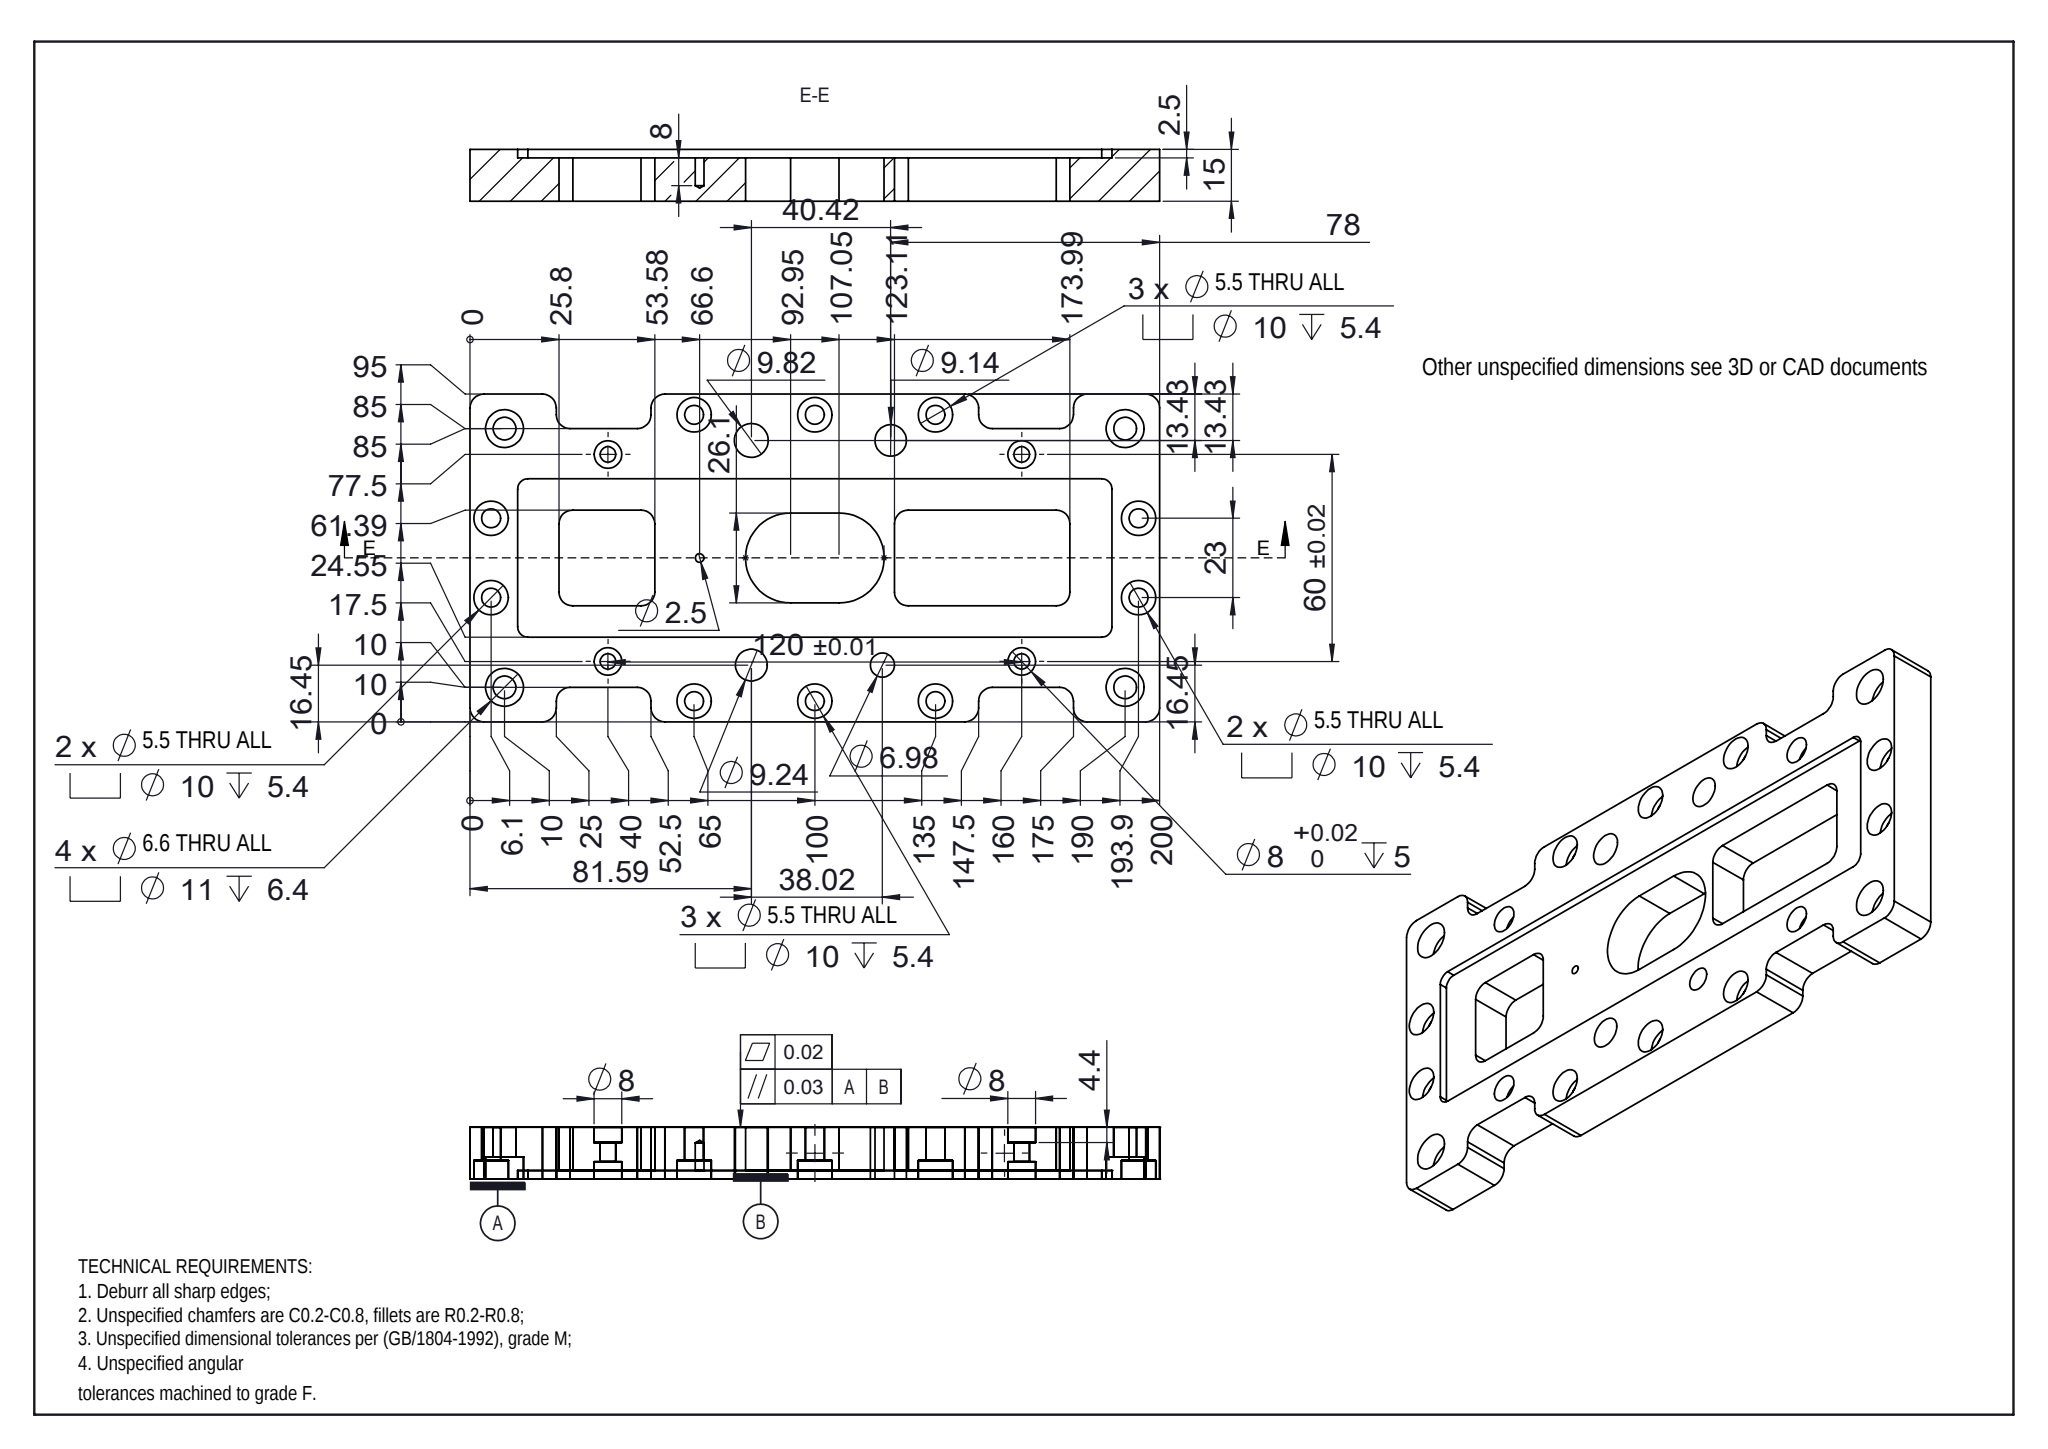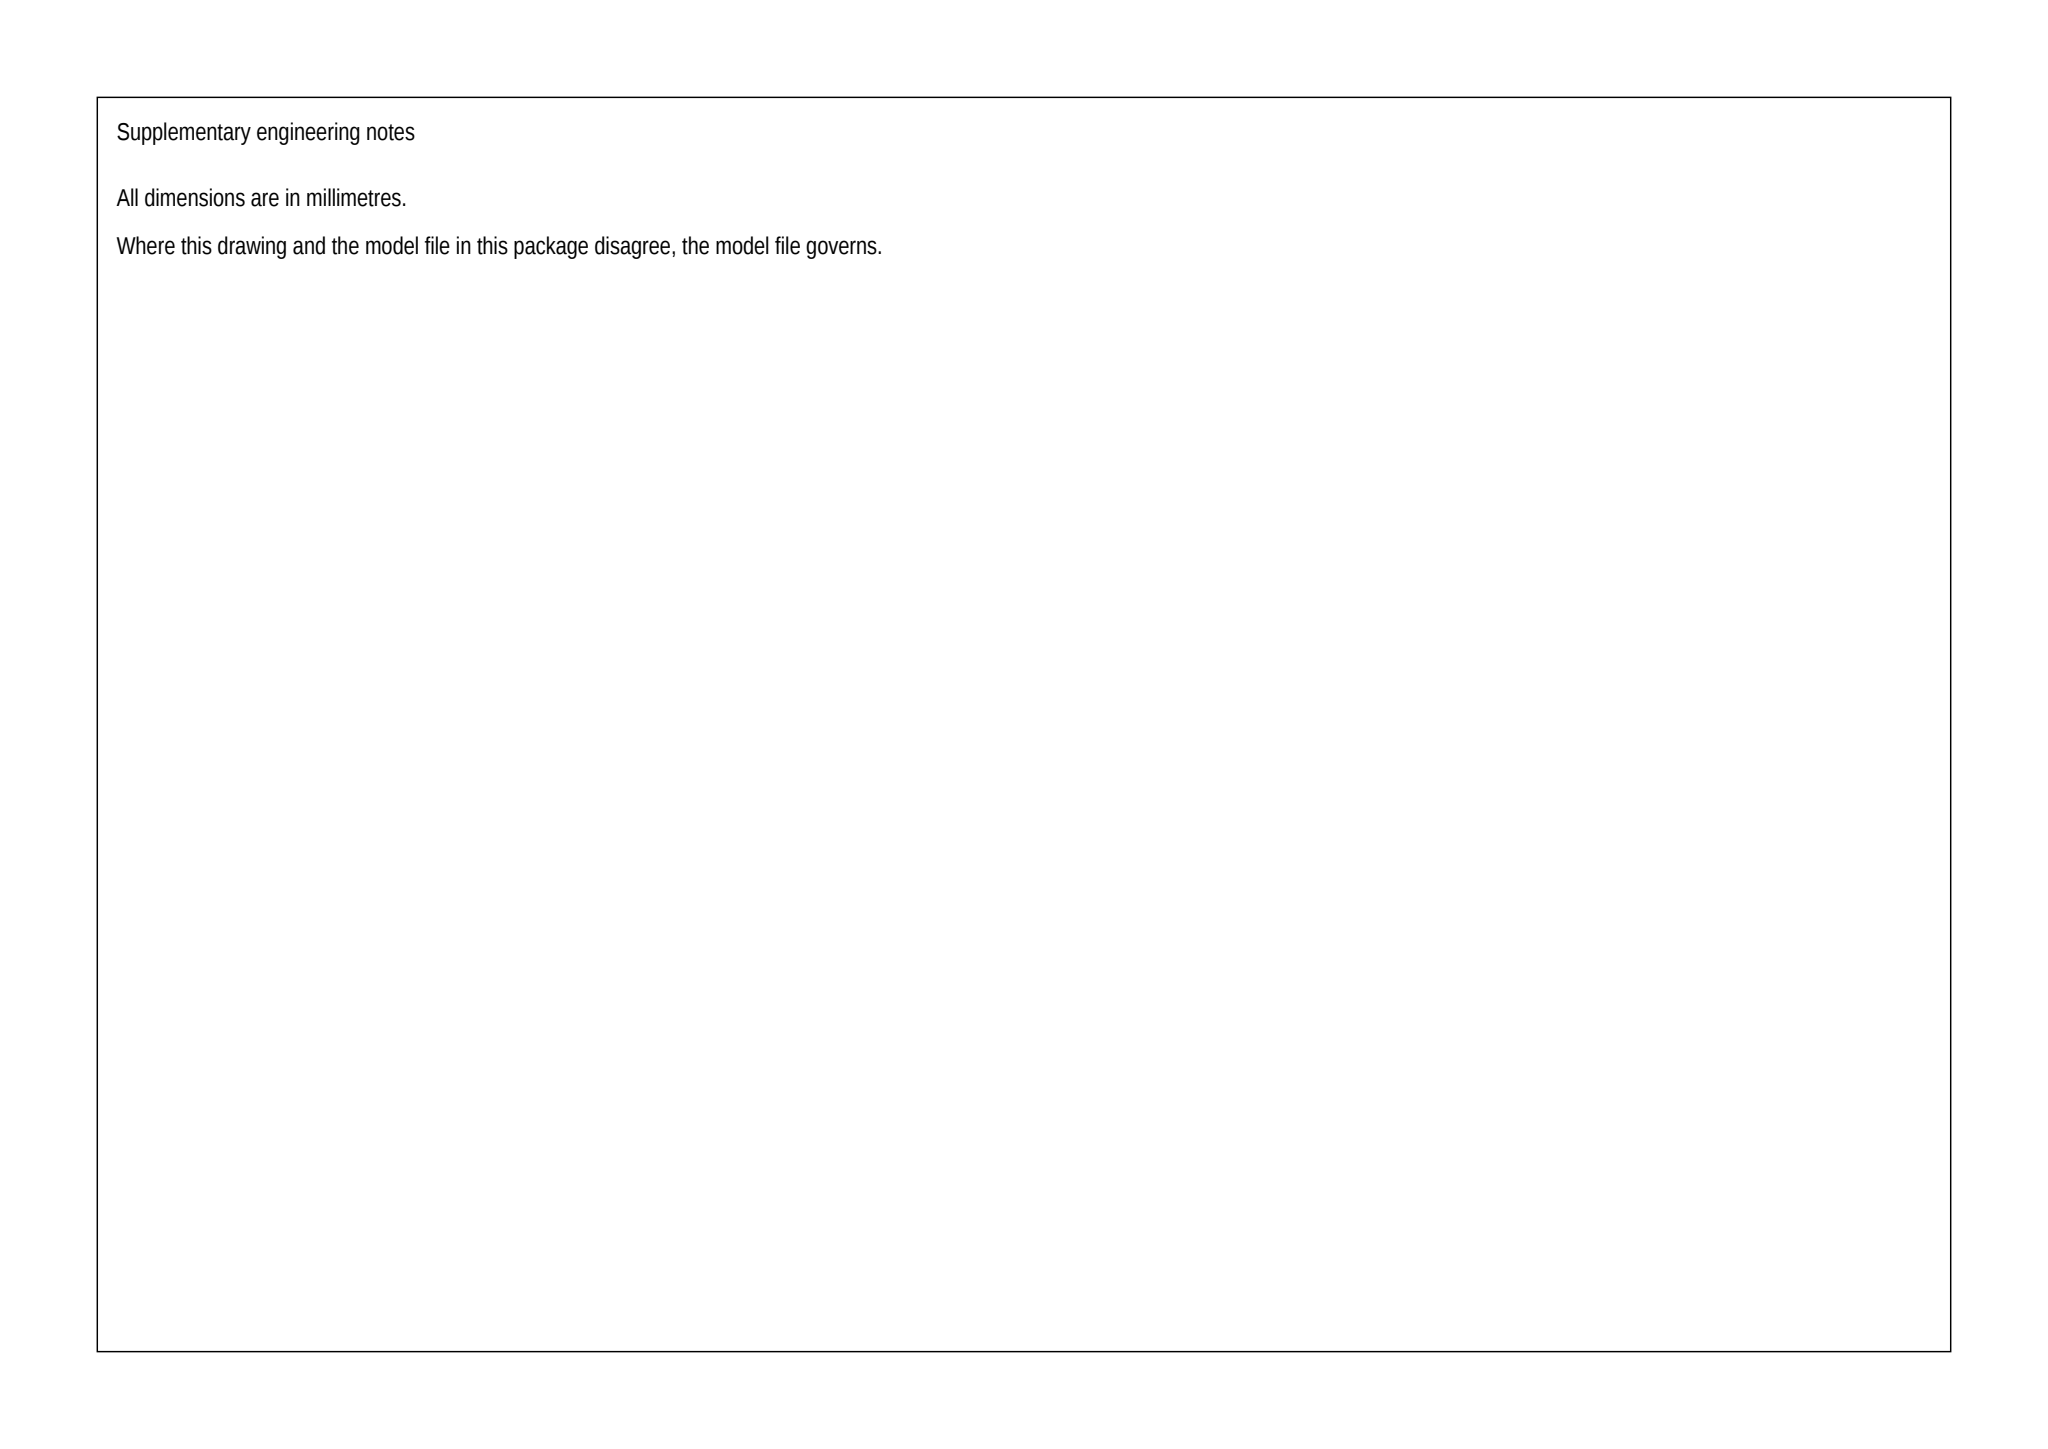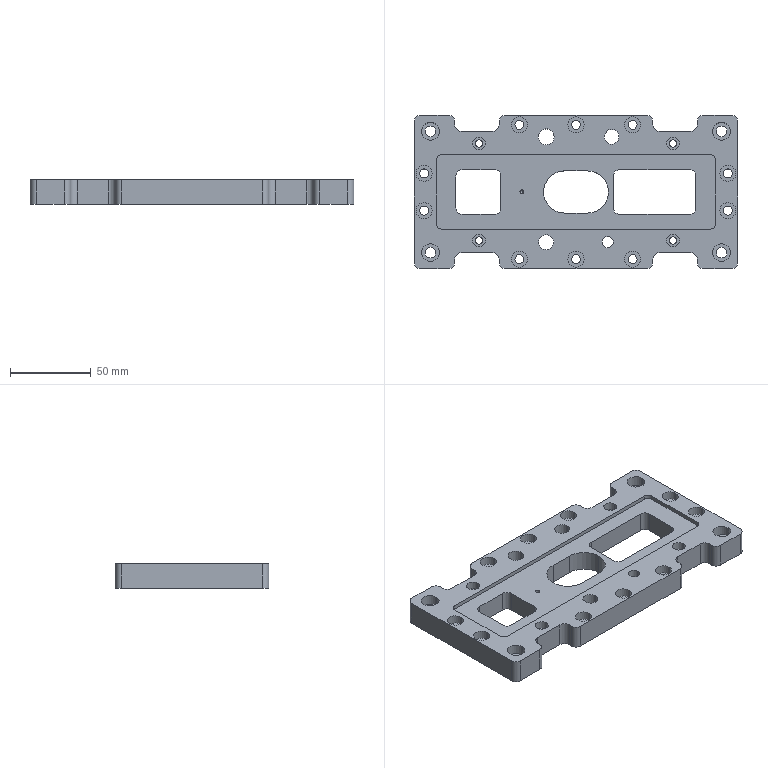Part | SolidWorks | mm | 1 solid | 186 faces | box 200 x 95 x 15 mm | volume 194152 mm3 | cylinder 125 | plane 59 | cone 2 | commonest cylinder face diameters 8 x44 10 x20 5.5 x20 11 x8 6.6 x8 4.5 x8 6 x4 26.1 x3
Drawing notes:
PLATE 200 X 95 X 15 THK, FLAT - NO BENT FLANGES/TABS, 4X CNR R4 | from the solid: bbox 200x95x15; all cyls axis z, only x/y/z planes, no fillets; Ø8 L15 at (4,4),(4,91),(196,4),(196,91)
TOP RECESS 172.4 X 45.9 DP 2.5, R3 CNRS, X13.8-186.2, Y24.55-70.45 | from the solid: x-planes 13.8/186.2, y-planes 24.55/70.45; Ø6 L2.5 at (16.8,27.55),(16.8,67.45),(183.2,27.55),(183.2,67.45)=R3; floor z=12.5
LH POCKET 27.78 SQ DP 12.5, R4 CNRS, X25.8-53.58, Y33.61-61.39 | from the solid: Ø8 L12.5 at (29.8,37.61),(29.8,57.39),(49.58,37.61),(49.58,57.39); planes x25.8/53.58, y33.61/61.39; floor z=2.5
RH POCKET 50.88 X 27.78 DP 12.5, R4 CNRS, X123.11-173.99, Y33.61-61.39 | from the solid: Ø8 L12.5 at (127.11,37.61),(127.11,57.39),(169.99,37.61),(169.99,57.39); planes x123.11/173.99, y33.61/61.39
CTR OBROUND 26.1 W X 40.2 LG DP 12.5, END CTRS X92.95 & X107.05, Y47.5 | from the solid: Ø26.1 L12.5 cyls at (92.95,47.5) and (107.05,47.5); 14.1 ctr dist + 26.1 = 40.2 lg
4X EDGE NOTCH 27.5 W X 10 DP THRU THK, R4 CNRS, X25-52.5 & 147.5-175, Y0 & Y95 | from the solid: y-planes 10(2)/85(2) between x25/52.5 and x147.5/175; Ø8 L15 at (29,6),(48.5,6),(151.5,6),(171,6) + y89 mirrors
NOTCH ENTRY RNDS R4 AT X21, 56.5, 143.5, 179, BOTH EDGES | from the solid: Ø8 L15 cyls at (21,4),(56.5,4),(143.5,4),(179,4) and y=91 mirrors
ALL PKT & CBORE DP FROM TOP FACE EXC Ø8 DP 4.4 FROM BOT FACE | from the solid: full faces z=0 and z=15; feature floors z=12.5,10.0,9.6,8.6 from top, 4.4 from bot
6X Ø5.5 THRU, CBORE Ø10 DP 5.4 FROM TOP FACE; AT X65, X100, X135 AND Y6 & Y89 FROM PLATE CORNER X0 Y0 | from the solid: cylinders [5.5,z,[65/100/135, 6 & 89],9.6] with [10.0,z,[65/100/135, 6 & 89],5.4]
4X Ø5.5 THRU, CBORE Ø10 DP 5.4 FROM TOP FACE; AT X6.1 & X193.9, Y36 & Y59 | from the solid: cylinders [5.5,z,[6.1 & 193.9, 36 & 59],9.6] with [10.0,z,[6.1 & 193.9, 36 & 59],5.4]
4X Ø6.6 THRU, CBORE Ø11 DP 6.4 FROM TOP FACE; AT X10 & X190, Y10 & Y85 | from the solid: cylinders [6.6,z,[10 & 190, 10 & 85],8.6] with [11.0,z,[10 & 190, 10 & 85],6.4]
Ø6.98 THRU 15 THK; CTR AT X119.6, Y16.5 FROM PLATE CORNER X0 Y0 | from the solid: hole/bore 6.98 axis z at (119.6,16.5) from 0.0 to 15.0
Ø2.5 HOLE, 8 DEEP (Z4.5 TO Z12.5, i.e. FROM RECESS FLOOR); CTR X66.6, Y47.5 FROM PLATE CORNER X0 Y0 | from the solid: cylinders: hole/bore dia 2.5, axis z at [66.6, 47.5], from 4.5 to 12.5
1X Ø8 +0.02/0 BORE DP 5 FROM TOP FACE (Z10 TO Z15); CTR X160, Y17.5 FROM PLATE CORNER X0 Y0 | from the solid: cylinders: hole/bore dia 8.0, axis z at [160.0, 17.5], from 10.0 to 15.0
POCKET/OBROUND FLOOR LEVEL: WALLS RUN Z0 TO Z12.5, i.e. 12.5 DEEP FROM THE 2.5 RECESS FLOOR (Z12.5), FLOOR AT Z0 = BOTTOM FACE LEVEL | from the solid: axis_planes x25.8 / x53.6 / x123.1 / x174.0 extent z [0.0, 12.5]; cylinders obround ends dia 26.1 at [93.0,47.5] & [107.1,47.5] from 0.0 to 12.5
4X Ø4.5 HOLE, Z4.4 TO Z10 (NOT THRU); CTRS X40 & X160, Y17.5 & Y77.5 FROM PLATE CORNER X0 Y0 | from the solid: cylinders: hole/bore Ø4.5 z from 4.4 to 10.0 at (40,17.5),(40,77.5),(160,17.5),(160,77.5)
1X Ø8 CBORE DP 4.4 FROM BOT FACE (Z0 TO Z4.4) AT X160, Y17.5 FROM PLATE CORNER X0 Y0 (ONE PLACE ONLY) | from the solid: cylinders: hole/bore Ø8 z from 0.0 to 4.4 at (160,17.5) — no other Ø8 bottom-face bore present
build123d program:
from build123d import *

# Parameters (mm, degrees)
SKETCH1_W                                       = 200
SKETCH1_H                                       = 95
BOSS_EXTRUDE1_DEPTH                             = 7.5
SKETCH2_W                                       = 50.88
SKETCH2_H                                       = 27.78
SKETCH2_W_2                                     = 27.78
CUT_EXTRUDE2_DEPTH                              = 112.72
SKETCH9_R                                       = 4
CUT_EXTRUDE6_DEPTH                              = 5
M4_HEX_SOCKET_HEAD_CAP_SCREW_CBORE1_D           = 4.5
M4_HEX_SOCKET_HEAD_CAP_SCREW_CBORE1_CBORE_D     = 8
M4_HEX_SOCKET_HEAD_CAP_SCREW_CBORE1_CBORE_DEPTH = 4.4
MIRROR2_COPY_1_SKETCH_R                         = 4
MIRROR2_COPY_1_DEPTH                            = 5
MIRROR2_COPY_2_D                                = 4.5
MIRROR2_COPY_2_CBORE_D                          = 8
MIRROR2_COPY_2_CBORE_DEPTH                      = 4.4
FILLET7_R                                       = 4
CUT_EXTRUDE7_DEPTH                              = 2.5
F_2_5_2_5_DIAMETER_HOLE1_D                      = 2.5
F_2_5_2_5_DIAMETER_HOLE1_DEPTH                  = 8
F_2_5_2_5_DIAMETER_HOLE1_TIP                    = 0.7511
M6_HEX_SOCKET_HEAD_CAP_SCREW_CBORE1_D           = 6.6
M6_HEX_SOCKET_HEAD_CAP_SCREW_CBORE1_CBORE_D     = 11
M6_HEX_SOCKET_HEAD_CAP_SCREW_CBORE1_CBORE_DEPTH = 6.4
M5_HEX_SOCKET_HEAD_CAP_SCREW_CBORE1_D           = 5.5
M5_HEX_SOCKET_HEAD_CAP_SCREW_CBORE1_CBORE_D     = 10
M5_HEX_SOCKET_HEAD_CAP_SCREW_CBORE1_CBORE_DEPTH = 5.4
CUT_EXTRUDE8_DEPTH                              = 112.72
FILLET8_R                                       = 4
MIRROR6_COPY_1_DEPTH                            = 112.72
FILLET9_R                                       = 4
FILLET10_R                                      = 4
M5_HEX_SOCKET_HEAD_CAP_SCREW_CBORE2_D           = 5.5
M5_HEX_SOCKET_HEAD_CAP_SCREW_CBORE2_CBORE_D     = 10
M5_HEX_SOCKET_HEAD_CAP_SCREW_CBORE2_CBORE_DEPTH = 5.4
SKETCH24_R                                      = 4.91
SKETCH24_R_2                                    = 4.621
SKETCH24_R_3                                    = 3.491
SKETCH24_R_4                                    = 4.57
CUT_EXTRUDE9_DEPTH                              = 42


with BuildPart() as part:
    # Sketch1 → Boss-Extrude1 (new, symmetric)
    with BuildSketch(Plane.XY):
        Rectangle(SKETCH1_W, SKETCH1_H)
    extrude(amount=BOSS_EXTRUDE1_DEPTH, both=True)

    # Sketch2 → Cut-Extrude2 (cut, through all)
    with BuildSketch(Plane.XY.offset(7.5)):
        with Locations((48.55, 0)):
            Rectangle(SKETCH2_W, SKETCH2_H)
        with Locations((-60.31, 0)):
            Rectangle(SKETCH2_W_2, SKETCH2_H)
        with BuildLine():
            Line((-7.05, 13.05), (7.05, 13.05))
            ThreePointArc((7.05, 13.05), (20.1, 0), (7.05, -13.05))
            Line((7.05, -13.05), (-7.05, -13.05))
            ThreePointArc((-7.05, -13.05), (-20.1, 0), (-7.05, 13.05))
        make_face()
    extrude(amount=-CUT_EXTRUDE2_DEPTH, mode=Mode.SUBTRACT)

    # Sketch9 → Cut-Extrude6 (cut)
    with BuildSketch(Plane.XY.offset(7.5)):
        with Locations((60, -30)):
            Circle(SKETCH9_R)
    cut_extrude6 = extrude(amount=-CUT_EXTRUDE6_DEPTH, mode=Mode.SUBTRACT)

    # M4 Hex Socket Head Cap Screw CBORE1 (through all)
    with Locations(Plane(origin=(0, 0, -7.5), x_dir=(-1, 0, 0), z_dir=(0, 0, -1))):
        with Locations((-60, -30)):
            m4_hex_socket_head_cap_screw_cbore1 = CounterBoreHole(M4_HEX_SOCKET_HEAD_CAP_SCREW_CBORE1_D / 2, M4_HEX_SOCKET_HEAD_CAP_SCREW_CBORE1_CBORE_D / 2, M4_HEX_SOCKET_HEAD_CAP_SCREW_CBORE1_CBORE_DEPTH)

    # Mirror1: Cut-Extrude6, M4 Hex Socket Head Cap Screw CBORE1 across plane
    add(cut_extrude6.mirror(Plane.ZX), mode=Mode.SUBTRACT)
    add(m4_hex_socket_head_cap_screw_cbore1.mirror(Plane.ZX), mode=Mode.SUBTRACT)

    # Mirror2: Cut-Extrude6, M4 Hex Socket Head Cap Screw CBORE1 across plane
    add(cut_extrude6.mirror(Plane(origin=(0, 0, 0), x_dir=(0, 0, 1), z_dir=(1, 0, 0))), mode=Mode.SUBTRACT)
    add(m4_hex_socket_head_cap_screw_cbore1.mirror(Plane(origin=(0, 0, 0), x_dir=(0, 0, 1), z_dir=(1, 0, 0))), mode=Mode.SUBTRACT)

    # Mirror2 copy 1 sketch → Mirror2 copy 1 (cut)
    with BuildSketch(Plane(origin=(0, 0, 7.5), x_dir=(-1, 0, 0), z_dir=(0, 0, 1))):
        with Locations((60, -30)):
            Circle(MIRROR2_COPY_1_SKETCH_R)
    extrude(amount=-MIRROR2_COPY_1_DEPTH, mode=Mode.SUBTRACT)

    # Mirror2 copy 2 (through all)
    with Locations(Plane(origin=(0, 0, -7.5), x_dir=(1, 0, 0), z_dir=(0, 0, -1))):
        with Locations((-60, -30)):
            CounterBoreHole(MIRROR2_COPY_2_D / 2, MIRROR2_COPY_2_CBORE_D / 2, MIRROR2_COPY_2_CBORE_DEPTH)

    # Fillet7
    fillet7_edges = [part.edges().sort_by_distance(p)[0] for p in [
        (-46.42, 13.89, 0),
        (-46.42, -13.89, 0),
        (-74.2, -13.89, 0),
        (-74.2, 13.89, 0),
        (23.11, 13.89, 0),
        (73.99, 13.89, 0),
        (73.99, -13.89, 0),
        (23.11, -13.89, 0),
    ]]
    fillet(fillet7_edges, radius=FILLET7_R)

    # Sketch12 → Cut-Extrude7 (cut)
    with BuildSketch(Plane.XY.offset(7.5)):
        with BuildLine():
            Line((83.2, 22.95), (-83.2, 22.95))
            ThreePointArc((-83.2, 22.95), (-85.321, 22.071), (-86.2, 19.95))
            Line((-86.2, 19.95), (-86.2, -19.95))
            ThreePointArc((-86.2, -19.95), (-85.321, -22.071), (-83.2, -22.95))
            Line((-83.2, -22.95), (83.2, -22.95))
            ThreePointArc((83.2, -22.95), (85.321, -22.071), (86.2, -19.95))
            Line((86.2, -19.95), (86.2, 19.95))
            ThreePointArc((86.2, 19.95), (85.321, 22.071), (83.2, 22.95))
        make_face()
    extrude(amount=-CUT_EXTRUDE7_DEPTH, mode=Mode.SUBTRACT)

    # 2.5 _2.5_ Diameter Hole1
    with Locations(Plane.XY.offset(5)):
        with Locations((-33.4, 0)):
            Hole(F_2_5_2_5_DIAMETER_HOLE1_D / 2, depth=F_2_5_2_5_DIAMETER_HOLE1_DEPTH)
            with Locations((0, 0, -(F_2_5_2_5_DIAMETER_HOLE1_DEPTH + F_2_5_2_5_DIAMETER_HOLE1_TIP / 2))):  # 118° drill point
                Cone(0, F_2_5_2_5_DIAMETER_HOLE1_D / 2, F_2_5_2_5_DIAMETER_HOLE1_TIP, mode=Mode.SUBTRACT)

    # M6 Hex Socket Head Cap Screw CBORE1 (through all)
    with Locations(Plane.XY.offset(7.5)):
        with Locations((-90, 37.5), (-90, -37.5), (90, 37.5), (90, -37.5)):
            CounterBoreHole(M6_HEX_SOCKET_HEAD_CAP_SCREW_CBORE1_D / 2, M6_HEX_SOCKET_HEAD_CAP_SCREW_CBORE1_CBORE_D / 2, M6_HEX_SOCKET_HEAD_CAP_SCREW_CBORE1_CBORE_DEPTH)

    # M5 Hex Socket Head Cap Screw CBORE1 (through all)
    with Locations(Plane.XY.offset(7.5)):
        with Locations((-35, -41.5), (0, -41.5), (35, -41.5)):
            m5_hex_socket_head_cap_screw_cbore1 = CounterBoreHole(M5_HEX_SOCKET_HEAD_CAP_SCREW_CBORE1_D / 2, M5_HEX_SOCKET_HEAD_CAP_SCREW_CBORE1_CBORE_D / 2, M5_HEX_SOCKET_HEAD_CAP_SCREW_CBORE1_CBORE_DEPTH)

    # Mirror3: M5 Hex Socket Head Cap Screw CBORE1 across plane
    add(m5_hex_socket_head_cap_screw_cbore1.mirror(Plane.ZX), mode=Mode.SUBTRACT)

    # Sketch21 → Cut-Extrude8 (cut, through all)
    with BuildSketch(Plane.XY.offset(7.5)):
        with BuildLine():
            Line((47.5, 47.5), (75, 47.5))
            Line((75, 47.5), (75, 41.5))
            ThreePointArc((75, 41.5), (73.828, 38.672), (71, 37.5))
            Line((71, 37.5), (51.5, 37.5))
            ThreePointArc((51.5, 37.5), (48.672, 38.672), (47.5, 41.5))
            Line((47.5, 41.5), (47.5, 47.5))
        make_face()
    cut_extrude8 = extrude(amount=-CUT_EXTRUDE8_DEPTH, mode=Mode.SUBTRACT)

    # Fillet8
    fillet8_edges = [part.edges().sort_by_distance(p)[0] for p in [
        (47.5, 47.5, 0),
        (75, 47.5, 0),
    ]]
    fillet(fillet8_edges, radius=FILLET8_R)

    # Mirror5: Cut-Extrude8 across plane
    add(cut_extrude8.mirror(Plane.ZX), mode=Mode.SUBTRACT)

    # Mirror6: Cut-Extrude8 across plane
    add(cut_extrude8.mirror(Plane(origin=(0, 0, 0), x_dir=(0, 0, 1), z_dir=(1, 0, 0))), mode=Mode.SUBTRACT)

    # Mirror6 copy 1 sketch → Mirror6 copy 1 (cut, through all)
    with BuildSketch(Plane(origin=(0, 0, 7.5), x_dir=(-1, 0, 0), z_dir=(0, 0, 1))):
        with BuildLine():
            Line((47.5, 47.5), (75, 47.5))
            Line((75, 47.5), (75, 41.5))
            ThreePointArc((75, 41.5), (73.828, 38.672), (71, 37.5))
            Line((71, 37.5), (51.5, 37.5))
            ThreePointArc((51.5, 37.5), (48.672, 38.672), (47.5, 41.5))
            Line((47.5, 41.5), (47.5, 47.5))
        make_face()
    extrude(amount=-MIRROR6_COPY_1_DEPTH, mode=Mode.SUBTRACT)

    # Fillet9
    fillet9_edges = [part.edges().sort_by_distance(p)[0] for p in [
        (47.5, -47.5, 0),
        (75, -47.5, 0),
        (-47.5, -47.5, 0),
        (-75, -47.5, 0),
        (-47.5, 47.5, 0),
        (-75, 47.5, 0),
    ]]
    fillet(fillet9_edges, radius=FILLET9_R)

    # Fillet10
    fillet10_edges = [part.edges().sort_by_distance(p)[0] for p in [
        (-100, 47.5, 0),
        (100, 47.5, 0),
        (100, -47.5, 0),
        (-100, -47.5, 0),
    ]]
    fillet(fillet10_edges, radius=FILLET10_R)

    # M5 Hex Socket Head Cap Screw CBORE2 (through all)
    with Locations(Plane.XY.offset(7.5)):
        with Locations((-93.9, 11.5), (-93.9, -11.5)):
            m5_hex_socket_head_cap_screw_cbore2 = CounterBoreHole(M5_HEX_SOCKET_HEAD_CAP_SCREW_CBORE2_D / 2, M5_HEX_SOCKET_HEAD_CAP_SCREW_CBORE2_CBORE_D / 2, M5_HEX_SOCKET_HEAD_CAP_SCREW_CBORE2_CBORE_DEPTH)

    # Mirror7: M5 Hex Socket Head Cap Screw CBORE2 across plane
    add(m5_hex_socket_head_cap_screw_cbore2.mirror(Plane(origin=(0, 0, 0), x_dir=(0, 0, 1), z_dir=(1, 0, 0))), mode=Mode.SUBTRACT)

    # Sketch24 → Cut-Extrude9 (cut)
    with BuildSketch(Plane.XY.offset(7.5)):
        with Locations((-18.412, 34.069)):
            Circle(SKETCH24_R)
        with Locations((-18.412, -31.047)):
            Circle(SKETCH24_R_2)
        with Locations((19.61, -31.047)):
            Circle(SKETCH24_R_3)
        with Locations((22.005, 34.069)):
            Circle(SKETCH24_R_4)
    extrude(amount=-CUT_EXTRUDE9_DEPTH, mode=Mode.SUBTRACT)


solid = part.part